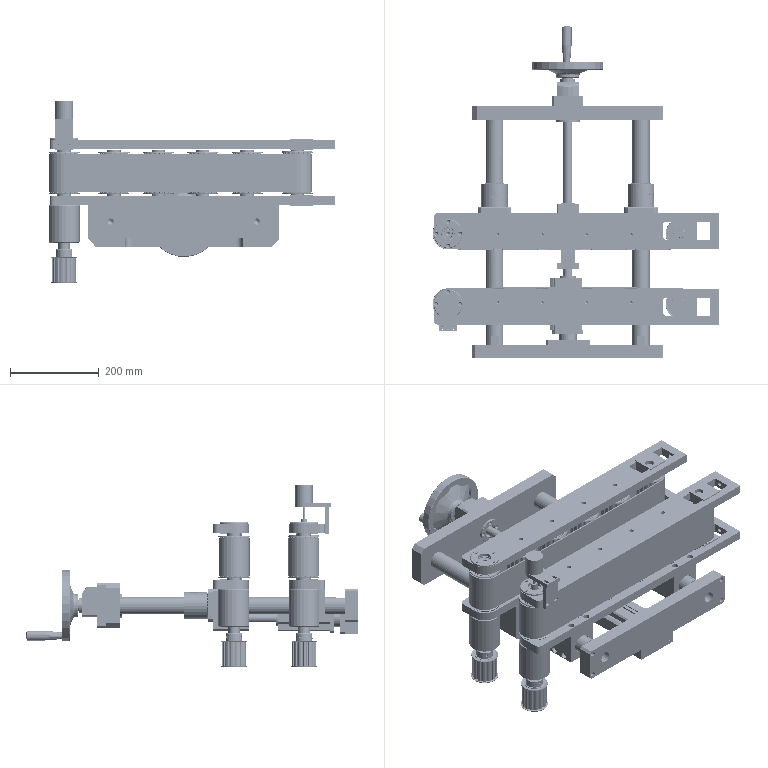Assembly | SolidWorks | mm | 131 component files | 548 solids | 15927 faces | box 646.6 x 748 x 409 mm | volume 15901574 mm3 | plane 6016 | cylinder 5265 | spline 3633 | cone 837 | torus 110 | sphere 66 | commonest cylinder face diameters 2.94 x548 2.84 x548 5.667 x216 58.13 x204 63.31 x192 0.361 x182 0.154 x168 0.628 x156
Bill of materials:
11_16X160 | 1 |  | Disc-shaped handwheel-like body: a flat circular rim with a recessed, scalloped (lobed) inner face that slopes conically down to a raised central hub. The hub has a through bore with a small keyway-like notch. A tapered cylindrical handle sticks out from the rim face, parallel to the axis.
1105_LMKPUU40 | 2 |  | Flanged cylindrical housing: a long round body with a square flange near one end. The flange has chamfered corners and four corner through-holes. The body has a large through bore. Small spherical elements are visible inside the bore, and a short stepped spigot sits on the far side of the flange.
ref7 | 1 |  | Ring-shaped rolling-element assembly: concentric inner and outer rings with a single row of spheres between them. The faces are open (no visible shields). The outer cylindrical surface is plain.
6004E-Z | 26 |  | Ring-shaped rolling-element assembly: inner and outer rings with a single row of spheres in the gap. Faces are open, and the outer edges are slightly rounded or faceted.
CounterMountingPlate | 1 |  | Thick rectangular plate with small chamfers on all four corners, one large central through-hole offset toward one end, and four small corner through-holes.
DigitalDisplay.0 | 1 |  | Block with two concave arc-shaped ends. A short cylindrical boss sticks out from one face and a smaller pin from the opposite face. The block has a through-hole and a chamfered edge.
E6B2-CWZ1XEncoder | 1 |  | Cylindrical body with a short smaller-diameter pilot step and a slender shaft coming out of one end. The shaft appears to have a flat along part of its length.
EncoderAxis | 1 |  | Stepped cylindrical pin: a larger central collar between two smaller shaft sections of different diameters. The end view shows flats or an irregular polygonal outline, and one end is lightly chamfered.
EncoderMountingSeat | 1 |  | L-shaped bracket. The horizontal plate has a rounded end with a large central hole and three small holes around it. Two slots sit near the bend, and the vertical leg has two further slots near its free end.
FixedSeat | 2 |  | Cube-like block with a large through bore. A narrow slit runs from the bore out to one edge, forming a split clamp. One face has four small holes, with countersunk/conical entries visible from the opposite face.
GuidePostMountingPlate | 1 | 1023 Carbon Steel Plate (SS) | Long rectangular bar with chamfered edges and a large through-hole near each end. The underside has a central recess/cutout between two end pads, and there is a small square window. Rows of small holes run on the top and side faces.
GuideSleeve | 2 |  | Plain thin-walled cylindrical tube with open ends, constant wall thickness, and no other features.
HandwheelEndCap | 1 |  | Thick flat annular disc (washer-like) with a single central through-hole and chamfered outer edges.
HandwheelMountingPlate | 1 |  | Elongated flat rectangular bar/plate with chamfered corners, a stepped (counterbored) central hole surrounded by four small holes in a cross pattern, and a counterbored hole near each end.
hexagon socket head cap screws gb | 4 |  | Cap-screw-shaped part: cylindrical head with hexagonal socket recess and rounded top edge, plain cylindrical shank with chamfered tip.
LimitingBlock | 1 |  | Rectangular hollow frame block with a square through-opening, chamfered outer corners, and a small hole through each side wall.
Nut | 1 |  | Long rectangular bar with a T-shaped cross-section (wider flange on one side) and a large round bore running lengthwise through it.
RisingBeltCylinderSeat | 1 |  | Two parallel rectangular plates of different size with chamfered corners, connected by a central cylindrical hub/spacer; each plate has four larger holes and four smaller corner holes.
RisingCylinderOutputPlate | 1 |  | Fork/U-shaped bracket block: base with two upright prongs forming a rectangular slot, a raised central tongue on one face, and three holes in the base (larger central hole, two side holes).
RisingCylinderSeatPlate | 1 |  | Rectangular prismatic block with two larger through-holes in one face and two small holes in an adjacent perpendicular face.
RisingGuidePost | 2 |  | Long slender cylindrical pin with a small axial hole at one end and a slight reduced-diameter step near that end.
Rolling bearings 51103 GB 301-1995 | 1 |  | Two identical flat annular rings (washers) stacked coaxially with a gap, and one circular row of equal-size spheres between them. The overall layout looks like a thrust ball bearing.
ScrewRod | 1 |  | Slender solid stepped cylindrical shaft with three diameters decreasing toward one end.
ScrewRodBearingEndCap | 1 |  | Thin flat annular ring/flange with a large central bore and four countersunk holes equally spaced on a circle.
ScrewRodFixingNut | 2 |  | Ring with a large central bore and four rectangular slots evenly spaced around the outer periphery, with chamfered edges (resembles a slotted round nut shape).
SDA50-80Cylinder | 1 |  | Prismatic body with a roughly square cross-section and chamfered corners, a through-hole at each of the four corners running the full length, and long slots on its side faces. One end face has a large circular recess, and a short cylindrical boss sticks out of the other end.
SDA50-80CylinderPiston | 1 |  | Solid round rod. One end is flat. The other end has a narrow ring-shaped groove close to the end face and a chamfer on the edge.
BearingPlate3 | 16 |  | Flat ring with a large central hole and chamfered edges on both faces.
S16-H12-01(SupportWheel) | 8 |  | Toothed cylindrical part with a flange at each end and a central through-bore. The outer surface has evenly spaced axial teeth/grooves, and the bore has an internal step.
SupportWheelAxis | 8 |  | Stepped cylindrical pin with a long main body, a short section of slightly smaller diameter, and a small-diameter spigot at one end. The larger end face has a small central hole with a conical bottom.
'-SynchronousBeltLength1260 | 2 |  | Thin-walled closed band with an obround (stadium-shaped) outline, open at both ends.
TensionAdjustmentBlock | 4 |  | Solid rectangular bar with three round through-holes in one long face: two larger holes near the ends and one smaller hole between them. The holes are not evenly spaced.
TensionBlock | 4 |  | Block with an I-shaped cross-section: wide top and bottom plates joined by a narrower central body. It has a large vertical through-hole near one corner and a small horizontal hole in one side face.
BearingPlate2 | 4 |  | Flat ring with a large central hole, square-edged with no visible chamfers.
S16-H12-01 | 2 |  | Toothed cylindrical part with a flange at each end and a central through-bore, with an internal step inside the bore. It looks the same as the part shown for unnamed part.
TractionDrivenWheelAxis | 2 |  | Solid cylindrical pin with a slightly larger diameter in the middle and short, slightly smaller-diameter sections at both ends, forming small shoulders. The end faces are flat with small chamfers.
S14H-H12-01(FrontWheel) | 2 |  | Toothed cylindrical part with a flange at each end and an extended cylindrical hub on one side. The central bore has one rectangular keyway, and the hub has at least two small radial holes.
S16-H12-01(DriveWheel) | 2 |  | Cylindrical body with axial teeth around the outside and a thin flange at each end, with a keyed through bore. It looks like a toothed pulley.
TractionDriveAxis | 2 |  | Long, thin stepped cylindrical pin or shaft. It has a larger-diameter upper section, a longer smaller-diameter lower section, and a short reduced stub at the top end with a small axial hole.
TractionDriveWheelBearingHousing | 2 |  | Thick-walled cylindrical housing with a large central bore. A shallow raised ring sits on the top face, the bore has an internal step, and four axial holes are evenly spaced around the bore.
TractionDriveWheelLimitSleeve | 2 |  | Plain thin-walled cylindrical tube or sleeve, roughly as long as its outer diameter.
TractionDriveWheelLimitSleeve2 | 2 |  | Short, thin-walled ring (spacer or collar shape) whose axial length is much smaller than its diameter.
TractionDriveWheelLimitSleeve3 | 2 |  | Short cylindrical sleeve or spacer with a thicker wall than the other plain tubes, with axial length about half its diameter.
TractionDriveWheelBearingEndCap | 2 |  | Thin circular flange plate with a large central through hole, four countersunk holes evenly spaced around it, and a shallow raised spigot or boss on one face.
TractionMachineBottomPlate | 1 |  | Rectangular bar or plate with chamfered corners. It has two larger through holes near the ends and four small holes near the corners.
WheelMountingPlateA | 1 |  | Long, flat arm plate. One end is rounded and carries a large through hole with four small holes around it. The other end has an open rectangular slot that forms two fork tines. Four holes are spaced in a line along the centerline.
WheelMountingPlateA-1 | 1 | 1023 Carbon Steel Plate (SS) | Long, flat arm plate like part-8, with a large hole and four small holes at the rounded end and a forked open slot at the other end, plus extra groups of holes along its length.
WheelMountingPlateB | 1 |  | Long, flat arm plate with a large hole and four small holes at the rounded end, four holes in a line along the centerline, and a forked open slot at the far end. It also has small holes in the side edge near the large hole.
WheelMountingPlateB-1 | 1 |  | Long, flat arm plate like part-10, with a large hole and four small holes at the rounded end and a forked open slot at the far end, plus four-hole groups near both ends.
Mates:
1. coincident | WheelMountingPlateA-1 face at (290.493, -53.411, 641) dir (0, 1, 0) | TensionBlock-1 face at (260.493, -53.411, 621) dir (0, -1, 0)
2. coincident | WheelMountingPlateA-1 face at (-24.507, -33.411, 621) dir (0, 0, -1) | TensionBlock-1 face at (260.493, -8.411, 621) dir (0, 0, 1)
3. coincident | WheelMountingPlateA-1 face at (290.493, -73.411, 621) dir (1, 0, 0) | TensionAdjustmentBlock-1 face at (290.493, -33.411, 631) dir (-1, 0, 0)
4. concentric | WheelMountingPlateA-1 face at (290.493, -3.411, 631) dir (1, 0, 0) r 3.4 | TensionAdjustmentBlock-1 face at (310.493, -3.411, 631) dir (1, 0, 0) r 7
5. concentric | WheelMountingPlateA-1 face at (290.493, -63.411, 631) dir (1, 0, 0) r 3.4 | TensionAdjustmentBlock-1 face at (310.493, -63.411, 631) dir (1, 0, 0) r 7
6. coincident | WheelMountingPlateB-1 face at (290.493, -244.411, 621) dir (1, 0, 0) | TensionAdjustmentBlock-2 face at (290.493, -204.411, 631) dir (-1, 0, 0)
7. coincident | WheelMountingPlateB-1 face at (290.493, -224.411, 641) dir (0, 1, 0) | TensionBlock-3 face at (260.493, -224.411, 641) dir (0, -1, 0)
8. concentric | WheelMountingPlateB-1 face at (290.493, -174.411, 631) dir (1, 0, 0) r 3.4 | TensionAdjustmentBlock-2 face at (310.493, -174.411, 631) dir (1, 0, 0) r 7
9. concentric | WheelMountingPlateB-1 face at (290.493, -234.411, 631) dir (1, 0, 0) r 3.4 | TensionAdjustmentBlock-2 face at (310.493, -234.411, 631) dir (1, 0, 0) r 7
10. concentric | TractionMachineBottomPlate-1 face at (-194.507, -319.411, 458) dir (0, 1, 0) r 20 | RisingGuidePost-1 face at (-194.507, 225.589, 458) dir (0, -1, 0) r 20
11. distance | TractionMachineBottomPlate-1 face at (-244.507, -319.411, 495.5) dir (0, -1, 0) | RisingGuidePost-1 face at (-194.507, -294.411, 458) dir (0, -1, 0)
12. concentric | TractionMachineBottomPlate-1 face at (135.493, -319.411, 458) dir (0, 1, 0) r 20 | RisingGuidePost-2 face at (135.493, 225.589, 458) dir (0, -1, 0) r 20
13. distance | TractionMachineBottomPlate-1 face at (-244.507, -319.411, 495.5) dir (0, -1, 0) | RisingGuidePost-2 face at (135.493, -294.411, 458) dir (0, -1, 0)
14. concentric | RisingGuidePost-1 face at (-194.507, 225.589, 458) dir (0, -1, 0) r 20 | FixedSeat-1 face at (-194.507, -244.411, 458) dir (0, 1, 0) r 20
15. parallel | TractionMachineBottomPlate-1 face at (-29.507, -304.411, 420.5) dir (0, 0, -1) | FixedSeat-1 face at (-194.507, -206.911, 423) dir (0, 0, -1)
16. concentric | RisingGuidePost-2 face at (135.493, 225.589, 458) dir (0, -1, 0) r 20 | FixedSeat-2 face at (135.493, -169.411, 458) dir (0, -1, 0) r 20
17. coincident | FixedSeat-1 face at (-194.507, -206.911, 423) dir (0, 0, -1) | FixedSeat-2 face at (135.493, -206.911, 423) dir (0, 0, -1)
18. coincident | TractionMachineBottomPlate-1 face at (-244.507, -289.411, 495.5) dir (0, 1, 0) | RisingBeltCylinderSeat-1 face at (-29.507, -289.411, 430.5) dir (0, -1, 0)
19. width | RisingBeltCylinderSeat-1 face at (20.493, -279.411, 393) dir (1, 0, 0) | RisingBeltCylinderSeat-1 face at (-79.507, -279.411, 393) dir (-1, 0, 0) | TractionMachineBottomPlate-1 face at (-244.507, -289.411, 495.5) dir (-1, 0, 0) | TractionMachineBottomPlate-1 face at (185.493, -289.411, 495.5) dir (1, 0, 0)
20. concentric | RisingGuidePost-2 face at (135.493, 225.589, 458) dir (0, -1, 0) r 20 | GuidePostMountingPlate-1 face at (135.493, -66.411, 458) dir (0, 1, 0) r 22
21. concentric | RisingGuidePost-1 face at (-194.507, 225.589, 458) dir (0, -1, 0) r 20 | GuidePostMountingPlate-1 face at (-194.507, -66.411, 458) dir (0, 1, 0) r 22
22. coincident | GuidePostMountingPlate-1 face at (-14.507, -69.411, 443) dir (0, 0, 1) | Nut-1 face at (-54.507, -104.411, 443) dir (0, 0, -1)
23. coincident | GuidePostMountingPlate-1 face at (-44.507, -69.411, 473) dir (1, 0, 0) | Nut-1 face at (-44.507, 30.589, 473) dir (-1, 0, 0)
24. width | RisingCylinderOutputPlate-1 face at (-57.007, -43.411, 468) dir (1, 0, 0) | RisingCylinderOutputPlate-1 face at (-2.007, -43.411, 468) dir (-1, 0, 0) | Nut-1 face at (-54.507, -104.411, 443) dir (-1, 0, 0) | Nut-1 face at (-4.507, -104.411, 443) dir (1, 0, 0)
25. coincident | GuidePostMountingPlate-1 face at (102.993, -28.411, 475) dir (0, -1, 0) | RisingCylinderOutputPlate-1 face at (-29.507, -28.411, 428) dir (0, 1, 0)
26. concentric | RisingGuidePost-1 face at (-194.507, 225.589, 458) dir (0, -1, 0) r 20 | HandwheelMountingPlate-1 face at (-194.507, 217.589, 458) dir (0, 1, 0) r 20
27. concentric | RisingGuidePost-2 face at (135.493, 225.589, 458) dir (0, -1, 0) r 20 | HandwheelMountingPlate-1 face at (135.493, 247.589, 458) dir (0, 1, 0) r 12
28. coincident | RisingGuidePost-2 face at (135.493, 225.589, 458) dir (0, 1, 0) | HandwheelMountingPlate-1 face at (135.493, 225.589, 458) dir (0, -1, 0)
29. coincident | WheelMountingPlateB-1 face at (-24.507, -204.411, 621) dir (0, 0, -1) | TensionBlock-3 face at (260.493, -179.411, 621) dir (0, 0, 1)
30. concentric | TensionBlock-3 face at (225.493, -197.911, 618.5) dir (0, 0, 1) r 9.5 | TractionDrivenWheel-1/6004E-Z-1 face at (225.493, -197.911, 527) dir (0, 0, 1) r 10
31. coincident | WheelMountingPlateB-1 plane at (225.493, -204.411, 631) dir (1, 0, 0) | TractionDrivenWheel-1/TractionDrivenWheelAxis-1 plane at (225.493, -197.911, 568.5) dir (-1, 0, 0)
32. coincident | 6004E-Z-1 face at (-299.852, -27.028, 624) dir (0, 0, -1) | TractionDriveWheelAssembly-1/TractionDriveAxis-1 face at (-299.507, -29.911, 624) dir (0, 0, 1)
33. concentric | 6004E-Z-1 face at (-299.507, -39.911, 630) dir (0, 0, -1) r 10 | TractionDriveWheelAssembly-1/TractionDriveAxis-1 face at (-299.507, -39.911, 965.247) dir (0, 0, 1) r 10
34. concentric | WheelMountingPlateB-1 face at (-299.507, -197.911, 641) dir (0, 0, -1) r 21 | 6004E-Z-2 face at (-299.507, -197.911, 631) dir (0, 0, 1) r 21
35. concentric | HandwheelMountingPlate-1 face at (-29.507, 217.589, 458) dir (0, 1, 0) r 10 | 11_16X160-1 face at (-29.507, 309.589, 458) dir (0, -1, 0) r 8
36. concentric | HandwheelMountingPlate-1 face at (-29.507, 217.589, 458) dir (0, 1, 0) r 10 | DigitalDisplay.0-1 face at (-29.507, 309.589, 458) dir (0, -1, 0) r 17
37. width | CounterMountingPlate-1 face at (-64.507, 269.589, 508) dir (0, 0, 1) | CounterMountingPlate-1 face at (-64.507, 269.589, 408) dir (0, 0, -1) | HandwheelMountingPlate-1 face at (185.493, 247.589, 408) dir (0, 0, -1) | HandwheelMountingPlate-1 face at (185.493, 247.589, 508) dir (0, 0, 1)
38. width | DigitalDisplay.0-1 face at (-53.507, 301.589, 437) dir (-1, 0, 0) | DigitalDisplay.0-1 face at (-5.507, 301.589, 437) dir (1, 0, 0) | CounterMountingPlate-1 face at (5.493, 269.589, 408) dir (1, 0, 0) | CounterMountingPlate-1 face at (-64.507, 269.589, 408) dir (-1, 0, 0)
39. coincident | 11_16X160-1 face at (-29.507, 309.589, 458) dir (0, -1, 0) | DigitalDisplay.0-1 face at (-29.507, 309.589, 458) dir (0, 1, 0)
40. concentric | ScrewRod-1 face at (-29.507, 267.589, 458) dir (0, -1, 0) r 8.35 | ScrewRodFixingNut-1 face at (-29.507, 255.589, 458) dir (0, -1, 0) r 8.5
41. coincident | HandwheelMountingPlate-1 face at (-29.507, 247.589, 458) dir (0, 1, 0) | CounterMountingPlate-1 face at (-29.507, 247.589, 458) dir (0, -1, 0)
42. coincident | DigitalDisplay.0-1 face at (-29.507, 269.589, 492.1) dir (0, -1, 0) | CounterMountingPlate-1 face at (-29.507, 269.589, 458) dir (0, 1, 0)
43. coincident | 11_16X160-1 face at (-32.409, 309.589, 447.806) dir (0.9992, 0, -0.03922) | ScrewRod-1 face at (-32.593, 304.589, 443.11) dir (0.9992, 0, -0.03922)
44. coincident | 11_16X160-1 face at (-30.585, 329.589, 430.521) dir (0, 1, 0) | HandwheelEndCap-1 face at (-29.507, 329.589, 458) dir (0, -1, 0)
45. concentric | ScrewRod-1 face at (-29.507, 327.589, 458) dir (0, 1, 0) r 2.5 | HandwheelEndCap-1 face at (-29.507, 329.589, 458) dir (0, 1, 0) r 3.5
46. concentric | ScrewRod-1 face at (-29.507, -441.983, 458) dir (0, -1, 0) r 10 | ScrewRodBearingEndCap-1 face at (-29.507, 217.589, 458) dir (0, -1, 0) r 14.5
47. coincident | HandwheelMountingPlate-1 face at (-29.507, 217.589, 458) dir (0, -1, 0) | ScrewRodBearingEndCap-1 face at (-29.507, 217.589, 458) dir (0, 1, 0)
48. concentric | HandwheelMountingPlate-1 face at (-29.507, 217.589, 479) dir (0, -1, 0) r 1.65 | ScrewRodBearingEndCap-1 face at (-29.507, 212.589, 479) dir (0, -1, 0) r 2.25
49. coincident | HandwheelMountingPlate-1 face at (-29.507, 238.589, 458) dir (0, 1, 0) | Rolling bearings 51103 GB 301-1995-1 face at (-37.584, 238.589, 454.031) dir (0, -1, 0)
50. concentric | HandwheelMountingPlate-1 face at (-29.507, 238.589, 458) dir (0, 1, 0) r 15 | Rolling bearings 51103 GB 301-1995-1 face at (-29.507, 234.363, 458) dir (0, -1, 0) r 8.5
51. coincident | Rolling bearings 51103 GB 301-1995-1 face at (-37.136, 247.589, 454.252) dir (0, 1, 0) | ScrewRodFixingNut-1 face at (-29.507, 247.589, 458) dir (0, -1, 0)
52. distance | ScrewRod-1 face at (-29.507, -82.411, 458) dir (0, -1, 0) | Nut-1 face at (-29.507, -119.411, 458) dir (0, -1, 0)
53. coincident | TractionMachineBottomPlate-1 face at (-29.507, -304.411, 420.5) dir (0, 0, -1) | RisingCylinderSeatPlate-1 face at (20.493, -289.411, 420.5) dir (0, 0, 1)
54. coincident | TractionMachineBottomPlate-1 face at (-244.507, -319.411, 495.5) dir (0, -1, 0) | RisingCylinderSeatPlate-1 face at (-29.507, -319.411, 406.75) dir (0, -1, 0)
55. width | RisingCylinderSeatPlate-1 face at (20.493, -289.411, 420.5) dir (1, 0, 0) | RisingCylinderSeatPlate-1 face at (-79.507, -289.411, 420.5) dir (-1, 0, 0) | TractionMachineBottomPlate-1 face at (-244.507, -289.411, 495.5) dir (-1, 0, 0) | TractionMachineBottomPlate-1 face at (185.493, -289.411, 495.5) dir (1, 0, 0)
56. concentric | RisingGuidePost-2 face at (135.493, 225.589, 458) dir (0, -1, 0) r 20 | 1105_LMKPUU40-1 face at (135.493, 47.467, 458) dir (0, 1, 0) r 30
57. coincident | GuidePostMountingPlate-1 face at (-232.007, 6.589, 400) dir (0, 1, 0) | 1105_LMKPUU40-1 face at (114.492, 6.589, 479.001) dir (0, -1, 0)
58. parallel | GuidePostMountingPlate-1 face at (172.993, -73.411, 400) dir (1, 0, 0) | 1105_LMKPUU40-1 face at (172.993, 6.589, 458) dir (1, 0, 0)
59. coincident | GuidePostMountingPlate-1 face at (135.493, -6.411, 458) dir (0, 1, 0) | GuideSleeve-1 face at (135.493, -6.411, 458) dir (0, 1, 0)
60. concentric | GuidePostMountingPlate-1 face at (135.493, -66.411, 458) dir (0, 1, 0) r 22 | GuideSleeve-1 face at (135.493, -6.411, 458) dir (0, -1, 0) r 22
61. coincident | Nut-1 face at (-54.507, -104.411, 473) dir (0, 0, 1) | LimitingBlock-1 face at (-44.507, 26.589, 473) dir (0, 0, -1)
62. coincident | Nut-1 face at (-14.507, 30.589, 473) dir (1, 0, 0) | LimitingBlock-1 face at (-14.507, 26.589, 443) dir (-1, 0, 0)
63. distance | Nut-1 face at (-29.507, 30.589, 458) dir (0, 1, 0) | LimitingBlock-1 face at (-29.507, 26.589, 458) dir (0, 1, 0)
64. coincident | FixedSeat-1 face at (-159.507, -244.411, 423) dir (0, -1, 0) | FixedSeat-2 face at (100.493, -244.411, 423) dir (0, -1, 0)
65. distance | GuidePostMountingPlate-1 face at (-232.007, -73.411, 400) dir (0, -1, 0) | FixedSeat-1 face at (-159.507, -169.411, 423) dir (0, 1, 0)
66. concentric | SDA50-80Cylinder-1 face at (-29.507, -205.411, 430.5) dir (0, 1, 0) r 10 | SDA50-80CylinderPiston-1 face at (-29.507, -149.411, 430.5) dir (0, 1, 0) r 10
67. distance | RisingCylinderOutputPlate-1 face at (-29.507, -43.411, 441.5) dir (0, 0, 1) | Nut-1 face at (-54.507, -104.411, 443) dir (0, 0, -1)
68. concentric | RisingCylinderOutputPlate-1 face at (-29.507, -28.411, 430.5) dir (0, 1, 0) r 5.5 | SDA50-80CylinderPiston-1 face at (-29.507, -149.411, 430.5) dir (0, 1, 0) r 10
69. coincident | RisingCylinderOutputPlate-1 face at (-29.507, -49.411, 430.5) dir (0, -1, 0) | SDA50-80CylinderPiston-1 face at (-29.507, -49.411, 430.5) dir (0, 1, 0)
70. concentric | RisingBeltCylinderSeat-1 face at (-53.507, -266.411, 406.5) dir (0, -1, 0) r 4.5 | SDA50-80Cylinder-1 face at (-53.507, -249.411, 406.5) dir (0, -1, 0) r 5.5
71. concentric | TensionAdjustmentBlock-1 face at (290.493, -39.911, 631) dir (1, 0, 0) r 4.1 | hexagon socket head cap screws gb-6 face at (304.493, -39.911, 631) dir (1, 0, 0) r 0.8
72. concentric | TensionAdjustmentBlock-2 face at (290.493, -197.911, 631) dir (1, 0, 0) r 4.1 | hexagon socket head cap screws gb-7 face at (304.493, -197.911, 631) dir (1, 0, 0) r 0.8
73. concentric | ScrewRodBearingEndCap-1 face at (-29.507, 217.589, 458) dir (0, -1, 0) r 27 | -6003-1 face at (-29.507, 231.299, 458) dir (0, 1, 0) r 17.5
74. coincident | ScrewRod-1 face at (-39.499, 217.589, 458.392) dir (0, 1, 0) | -6003-1 face at (-12.007, 217.589, 458) dir (0, -1, 0)
75. coincident | HandwheelMountingPlate-1 face at (-29.507, 227.589, 458) dir (0, -1, 0) | -6003-1 face at (-12.007, 227.589, 458) dir (0, 1, 0)
76. coincident | ScrewRodFixingNut-1 face at (-29.507, 255.589, 458) dir (0, 1, 0) | ScrewRodFixingNut-6 face at (-29.507, 255.589, 458) dir (0, -1, 0)
77. concentric | ScrewRod-1 face at (-29.507, 267.589, 458) dir (0, -1, 0) r 8.35 | ScrewRodFixingNut-6 face at (-29.507, 263.589, 458) dir (0, -1, 0) r 8.5
78. distance | EncoderAxis-1 face at (-293.716, -193.145, 654) dir (0, 0, 1) | TractionDriveWheelAssembly-2/TractionDriveAxis-1 face at (-299.507, -197.911, 636) dir (0, 0, 1)
79. concentric | TractionDriveWheelAssembly-2/TractionDriveAxis-1 face at (-299.507, -197.911, 636) dir (0, 0, 1) r 5 | EncoderAxis-1 face at (-299.507, -197.911, 814.656) dir (0, 0, 1) r 5
80. concentric | E6B2-CWZ1XEncoder-1 face at (-299.507, -182.911, 690) dir (0, 0, -1) r 1.25 | EncoderMountingSeat-1 face at (-299.507, -182.911, 683) dir (0, 0, -1) r 3.5
81. concentric | E6B2-CWZ1XEncoder-1 face at (-286.516, -205.411, 690) dir (0, 0, -1) r 1.25 | EncoderMountingSeat-1 face at (-286.516, -205.411, 683) dir (0, 0, -1) r 3.5
82. coincident | E6B2-CWZ1XEncoder-1 face at (-299.507, -197.911, 690) dir (0, 0, -1) | EncoderMountingSeat-1 face at (-299.507, -197.911, 690) dir (0, 0, 1)
83. distance | TensionBlock-1 face at (210.493, -58.411, 618.5) dir (-1, 0, 0) | WheelMountingPlateA-1 face at (185.493, -13.411, 641) dir (1, 0, 0)
84. coincident | TensionAdjustmentBlock-1 face at (310.493, -33.411, 631) dir (1, 0, 0) | hexagon socket head cap screws gb-6 face at (310.493, -39.911, 631) dir (-1, 0, 0)
85. coincident | WheelMountingPlateA-1-1 plane at (-24.507, -33.411, 505) dir (0, 1, 0) | GuidePostMountingPlate-1 plane at (-29.507, -33.411, 447.5) dir (0, 1, 0)
86. coincident | WheelMountingPlateA-1-1 face at (-24.507, -33.411, 495) dir (0, 0, -1) | GuidePostMountingPlate-1 face at (-29.507, -33.411, 495) dir (0, 0, 1)
87. concentric | WheelMountingPlateA-1-1 face at (82.993, -8.411, 515) dir (0, 0, 1) r 5.5 | GuidePostMountingPlate-1 face at (82.993, -8.411, 495) dir (0, 0, 1) r 4.25
88. concentric | WheelMountingPlateA-1-1 face at (-299.507, -39.911, 515) dir (0, 0, -1) r 23 | TractionDriveWheelAssembly-1/TractionDriveWheelLimitSleeve-1 face at (-299.507, -39.911, 520) dir (0, 0, -1) r 15
89. coincident | WheelMountingPlateA-1-1 face at (-24.507, -33.411, 495) dir (0, 0, -1) | TractionDriveWheelAssembly-1/TractionDriveWheelBearingHousing-2 face at (-320.507, -39.911, 495) dir (0, 0, 1)
90. coincident | WheelMountingPlateA-1 plane at (-24.507, -33.411, 631) dir (-1, 0, 0) | WheelMountingPlateA-1-1 plane at (-24.507, -33.411, 505) dir (-1, 0, 0)
91. coincident | WheelMountingPlateA-1 plane at (-24.507, -33.411, 631) dir (0, 1, 0) | WheelMountingPlateA-1-1 plane at (-24.507, -33.411, 505) dir (0, 1, 0)
92. distance | WheelMountingPlateA-1 face at (-24.507, -33.411, 641) dir (0, 0, 1) | WheelMountingPlateA-1-1 face at (-24.507, -33.411, 495) dir (0, 0, -1)
93. concentric | WheelMountingPlateA-1 face at (-299.507, -12.911, 621) dir (0, 0, -1) r 1.65 | TractionDriveWheelBearingEndCap-1 face at (-299.507, -12.911, 646) dir (0, 0, 1) r 2.25
94. concentric | WheelMountingPlateA-1 face at (-299.507, -66.911, 621) dir (0, 0, -1) r 1.65 | TractionDriveWheelBearingEndCap-1 face at (-299.507, -66.911, 646) dir (0, 0, 1) r 2.25
95. coincident | WheelMountingPlateA-1 face at (-24.507, -33.411, 641) dir (0, 0, 1) | TractionDriveWheelBearingEndCap-1 face at (-299.507, -7.411, 641) dir (0, 0, -1)
96. coincident | WheelMountingPlateA-1-1 face at (290.493, -13.411, 515) dir (0, -1, 0) | TensionBlock-7 face at (260.493, -13.411, 495) dir (0, 1, 0)
97. width | TensionBlock-7 face at (235.493, -33.411, 492.5) dir (0, 0, -1) | TensionBlock-7 face at (235.493, -33.411, 517.5) dir (0, 0, 1) | WheelMountingPlateA-1-1 face at (-24.507, -33.411, 515) dir (0, 0, 1) | WheelMountingPlateA-1-1 face at (-24.507, -33.411, 495) dir (0, 0, -1)
98. coincident | TensionBlock-1 face at (260.493, -58.411, 618.5) dir (1, 0, 0) | TensionBlock-7 face at (260.493, -58.411, 492.5) dir (1, 0, 0)
99. concentric | WheelMountingPlateA-1-1 face at (290.493, -3.411, 505) dir (1, 0, 0) r 3.4 | TensionAdjustmentBlock-5 face at (310.493, -3.411, 505) dir (1, 0, 0) r 7
100. concentric | WheelMountingPlateA-1-1 face at (290.493, -63.411, 505) dir (1, 0, 0) r 3.4 | TensionAdjustmentBlock-5 face at (310.493, -63.411, 505) dir (1, 0, 0) r 4.5
101. coincident | WheelMountingPlateA-1-1 face at (290.493, -73.411, 495) dir (1, 0, 0) | TensionAdjustmentBlock-5 face at (290.493, -33.411, 505) dir (-1, 0, 0)
102. concentric | TensionAdjustmentBlock-5 face at (290.493, -39.911, 505) dir (1, 0, 0) r 4.1 | hexagon socket head cap screws gb-8 face at (304.493, -39.911, 505) dir (1, 0, 0) r 0.8
103. coincident | TensionAdjustmentBlock-5 face at (310.493, -33.411, 505) dir (1, 0, 0) | hexagon socket head cap screws gb-8 face at (310.493, -39.911, 505) dir (-1, 0, 0)
104. concentric | TractionDrivenWheel-2/TractionDrivenWheelAxis-1 face at (225.493, -39.911, 520) dir (0, 0, -1) r 9.5 | TensionBlock-7 face at (225.493, -39.911, 517.5) dir (0, 0, -1) r 9.5
105. coincident | TractionDrivenWheel-2/BearingPlate2-2 face at (225.493, -39.911, 517.5) dir (0, 0, -1) | TensionBlock-7 face at (235.493, -33.411, 517.5) dir (0, 0, 1)
106. concentric | WheelMountingPlateA-1-1 face at (-187.007, -42.411, 495) dir (0, 0, -1) r 6 | SupportWheelAssembly-2/SupportWheelAxis-1 face at (-187.007, -42.411, 496) dir (0, 0, 1) r 6
107. concentric | WheelMountingPlateA-1-1 face at (112.993, -42.411, 495) dir (0, 0, -1) r 6 | SupportWheelAssembly-2/SupportWheelAxis-4 face at (112.993, -42.411, 496) dir (0, 0, 1) r 6
108. coincident | WheelMountingPlateA-1-1 face at (-24.507, -33.411, 515) dir (0, 0, 1) | SupportWheelAssembly-2/BearingPlate3-4 face at (112.993, -42.411, 515) dir (0, 0, -1)
109. coincident | TensionAdjustmentBlock-2 face at (310.493, -204.411, 631) dir (1, 0, 0) | hexagon socket head cap screws gb-7 face at (310.493, -197.911, 631) dir (-1, 0, 0)
110. distance | FixedSeat-1 face at (-159.507, -244.411, 423) dir (0, -1, 0) | TractionMachineBottomPlate-1 face at (-244.507, -289.411, 495.5) dir (0, 1, 0)
111. concentric | WheelMountingPlateB-1-1 face at (-218.507, -178.911, 515) dir (0, 0, 1) r 4.5 | FixedSeat-1 face at (-218.507, -178.911, 495) dir (0, 0, 1) r 3.4
112. concentric | WheelMountingPlateB-1-1 face at (-170.507, -178.911, 515) dir (0, 0, 1) r 4.5 | FixedSeat-1 face at (-170.507, -178.911, 495) dir (0, 0, 1) r 3.4
113. coincident | WheelMountingPlateB-1-1 face at (-24.507, -204.411, 495) dir (0, 0, -1) | FixedSeat-1 face at (-194.507, -206.911, 495) dir (0, 0, 1)
114. concentric | WheelMountingPlateB-1-1 face at (-299.507, -197.911, 515) dir (0, 0, -1) r 22.5 | TractionDriveWheelAssembly-2/TractionDriveWheelLimitSleeve-1 face at (-299.507, -197.911, 520) dir (0, 0, -1) r 15
115. coincident | WheelMountingPlateB-1-1 face at (-24.507, -204.411, 495) dir (0, 0, -1) | TractionDriveWheelAssembly-2/TractionDriveWheelBearingHousing-2 face at (-299.507, -176.911, 495) dir (0, 0, 1)
116. concentric | WheelMountingPlateB-1-1 face at (-299.507, -169.911, 515) dir (0, 0, 1) r 2.5 | TractionDriveWheelAssembly-2/TractionDriveWheelBearingHousing-2 face at (-299.507, -169.911, 410) dir (0, 0, -1) r 3.5
117. concentric | WheelMountingPlateA-1-1 face at (-299.507, -11.911, 515) dir (0, 0, 1) r 2.5 | TractionDriveWheelAssembly-1/TractionDriveWheelBearingHousing-2 face at (-299.507, -11.911, 410) dir (0, 0, -1) r 3.5
118. coincident | WheelMountingPlateB-1 plane at (-24.507, -204.411, 631) dir (-1, 0, 0) | WheelMountingPlateB-1-1 plane at (-24.507, -204.411, 505) dir (-1, 0, 0)
119. coincident | WheelMountingPlateB-1 plane at (-24.507, -204.411, 631) dir (0, 1, 0) | WheelMountingPlateB-1-1 plane at (-24.507, -204.411, 505) dir (0, 1, 0)
120. distance | WheelMountingPlateB-1 face at (-24.507, -204.411, 641) dir (0, 0, 1) | WheelMountingPlateB-1-1 face at (-24.507, -204.411, 495) dir (0, 0, -1)
121. concentric | WheelMountingPlateB-1 face at (-299.507, -170.911, 621) dir (0, 0, -1) r 1.65 | TractionDriveWheelBearingEndCap-2 face at (-299.507, -170.911, 646) dir (0, 0, 1) r 2.25
122. concentric | WheelMountingPlateB-1 face at (-299.507, -224.911, 621) dir (0, 0, -1) r 1.65 | TractionDriveWheelBearingEndCap-2 face at (-299.507, -224.911, 646) dir (0, 0, 1) r 2.25
123. coincident | WheelMountingPlateB-1 face at (-24.507, -204.411, 641) dir (0, 0, 1) | TractionDriveWheelBearingEndCap-2 face at (-267.007, -197.911, 641) dir (0, 0, -1)
124. concentric | E6B2-CWZ1XEncoder-1 face at (-299.507, -197.911, 690) dir (0, 0, 1) r 20 | EncoderAxis-1 face at (-299.507, -197.911, 814.656) dir (0, 0, 1) r 3
125. coincident | E6B2-CWZ1XEncoder-1 face at (-299.507, -197.911, 670) dir (0, 0, -1) | EncoderAxis-1 face at (-297.19, -196.005, 670) dir (0, 0, 1)
126. coincident | WheelMountingPlateB-1 face at (-339.507, -244.411, 621) dir (0, -1, 0) | EncoderMountingSeat-1 face at (-279.507, -244.411, 620) dir (0, 1, 0)
127. coincident | TensionBlock-3 face at (235.493, -204.411, 618.5) dir (0, 0, -1) | TractionDrivenWheel-1/BearingPlate2-2 face at (225.493, -197.911, 618.5) dir (0, 0, 1)
128. concentric | WheelMountingPlateB-1-1 face at (-187.007, -195.411, 495) dir (0, 0, -1) r 6 | SupportWheelAssembly-1/SupportWheelAxis-1 face at (-187.007, -195.411, 496) dir (0, 0, 1) r 6
129. concentric | WheelMountingPlateB-1-1 face at (112.993, -195.411, 495) dir (0, 0, -1) r 6 | SupportWheelAssembly-1/SupportWheelAxis-4 face at (112.993, -195.411, 496) dir (0, 0, 1) r 6
130. coincident | WheelMountingPlateB-1-1 face at (-24.507, -204.411, 515) dir (0, 0, 1) | SupportWheelAssembly-1/BearingPlate3-4 face at (112.993, -195.411, 515) dir (0, 0, -1)
131. coincident | WheelMountingPlateB-1-1 face at (290.493, -184.411, 515) dir (0, -1, 0) | TensionBlock-8 face at (260.493, -184.411, 515) dir (0, 1, 0)
132. width | TensionBlock-8 face at (235.493, -204.411, 492.5) dir (0, 0, -1) | TensionBlock-8 face at (235.493, -204.411, 517.5) dir (0, 0, 1) | WheelMountingPlateB-1-1 face at (-24.507, -204.411, 515) dir (0, 0, 1) | WheelMountingPlateB-1-1 face at (-24.507, -204.411, 495) dir (0, 0, -1)
133. coincident | TensionBlock-3 face at (260.493, -179.411, 643.5) dir (1, 0, 0) | TensionBlock-8 face at (260.493, -179.411, 517.5) dir (1, 0, 0)
134. concentric | WheelMountingPlateB-1-1 face at (290.493, -174.411, 505) dir (1, 0, 0) r 3.4 | TensionAdjustmentBlock-6 face at (310.493, -174.411, 505) dir (1, 0, 0) r 7
135. concentric | WheelMountingPlateB-1-1 face at (290.493, -234.411, 505) dir (1, 0, 0) r 3.4 | TensionAdjustmentBlock-6 face at (310.493, -234.411, 505) dir (1, 0, 0) r 7
136. coincident | WheelMountingPlateB-1-1 face at (290.493, -244.411, 495) dir (1, 0, 0) | TensionAdjustmentBlock-6 face at (290.493, -204.411, 505) dir (-1, 0, 0)
137. concentric | TensionAdjustmentBlock-6 face at (290.493, -197.911, 505) dir (1, 0, 0) r 4.1 | hexagon socket head cap screws gb-9 face at (304.493, -197.911, 505) dir (1, 0, 0) r 0.8
138. coincident | TensionAdjustmentBlock-6 face at (310.493, -204.411, 505) dir (1, 0, 0) | hexagon socket head cap screws gb-9 face at (310.493, -197.911, 505) dir (-1, 0, 0)
139. coincident | RisingBeltCylinderSeat-1 face at (-29.507, -256.411, 430.5) dir (0, 1, 0) | SDA50-80Cylinder-1 face at (6.465, -256.411, 600.874) dir (0, -1, 0)
140. coincident | TractionDriveWheelBearingEndCap-2 face at (-278.507, -197.911, 637) dir (0, 0, -1) | 6004E-Z-2 face at (-280.981, -201.393, 637) dir (0, 0, 1)
141. concentric | SupportWheelAxis-1 face at (-6.386, 0.2376, 181) dir (0, 0, -1) r 10 | BearingPlate3-1 face at (-6.386, 0.2376, 81) dir (0, 0, -1) r 10.1
142. coincident | SupportWheelAxis-1 face at (-6.386, 0.2376, 76) dir (0, 0, -1) | BearingPlate3-1 face at (-6.386, 0.2376, 76) dir (0, 0, -1)
143. concentric | SupportWheelAxis-1 face at (-6.386, 0.2376, 181) dir (0, 0, -1) r 10 | S16-H12-01(SupportWheel)-1 face at (-6.386, 0.2376, 81) dir (0, 0, 1) r 17.5
144. concentric | S16-H12-01(SupportWheel)-1 face at (-6.386, 0.2376, 93) dir (0, 0, -1) r 21 | 6004E-Z-1 face at (-6.386, 0.2376, 87) dir (0, 0, 1) r 21
145. coincident | S16-H12-01(SupportWheel)-1 face at (-6.386, 0.2376, 93) dir (0, 0, -1) | 6004E-Z-1 face at (-6.386, 13.125, 93) dir (0, 0, 1)
146. coincident | BearingPlate3-1 face at (-6.386, 0.2376, 81) dir (0, 0, 1) | 6004E-Z-1 face at (-6.386, 14.088, 81) dir (0, 0, -1)
147. concentric | SupportWheelAxis-1 face at (-6.386, 0.2376, 181) dir (0, 0, -1) r 10 | 6004E-Z-5 face at (-6.386, 0.2376, 170) dir (0, 0, -1) r 21
148. coincident | S16-H12-01(SupportWheel)-1 face at (-6.386, 0.2376, 164) dir (0, 0, 1) | 6004E-Z-5 face at (-1.45, -11.667, 164) dir (0, 0, -1)
149. concentric | SupportWheelAxis-1 face at (-6.386, 0.2376, 181) dir (0, 0, -1) r 10 | BearingPlate3-5 face at (-6.386, 0.2376, 181) dir (0, 0, -1) r 15.1
150. coincident | 6004E-Z-5 face at (-1.081, -12.556, 176) dir (0, 0, 1) | BearingPlate3-5 face at (-6.386, 0.2376, 176) dir (0, 0, -1)
151. coincident | -SynchronousBeltLength1260-1 plane at (143.614, -2.262, 128.5) dir (1, 0, 0) | SupportWheelAssembly plane at (143.614, 0, 0) dir (1, 0, 0)
152. coincident | SupportWheelAxis-1 plane at (-6.386, 0.2376, 128.5) dir (0, 1, 0) | -SynchronousBeltLength1260-1 plane at (-118.886, 0.2376, 128.5) dir (0, -1, 0)
153. coincident | SupportWheelAxis-1 plane at (-6.386, 0.2376, 128.5) dir (0, 0, 1) | -SynchronousBeltLength1260-1 plane at (-118.886, -2.262, 128.5) dir (0, 0, -1)
154. concentric | S16-H12-01-1 face at (-27.031, -1.559, 128) dir (0, 0, 1) r 21 | 6004E-Z-1 face at (-27.031, -1.559, 134) dir (0, 0, -1) r 21
155. coincident | S16-H12-01-1 face at (-27.031, -1.559, 128) dir (0, 0, 1) | 6004E-Z-1 face at (-27.376, 11.323, 128) dir (0, 0, -1)
156. coincident | S16-H12-01-1 face at (-27.031, -1.559, 57) dir (0, 0, -1) | 6004E-Z-2 face at (-31.646, 10.473, 57) dir (0, 0, 1)
157. concentric | S16-H12-01-1 face at (-27.031, -1.559, 57) dir (0, 0, -1) r 21 | 6004E-Z-2 face at (-27.031, -1.559, 51) dir (0, 0, 1) r 21
158. concentric | 6004E-Z-1 face at (-27.031, -1.559, 134) dir (0, 0, -1) r 10 | TractionDrivenWheelAxis-1 face at (-27.031, -1.559, 25) dir (0, 0, 1) r 10
159. coincident | 6004E-Z-1 face at (-27.402, 12.286, 140) dir (0, 0, 1) | TractionDrivenWheelAxis-1 face at (-27.031, -1.559, 140) dir (0, 0, 1)
160. coincident | 6004E-Z-1 face at (-27.402, 12.286, 140) dir (0, 0, 1) | BearingPlate2-1 face at (-27.031, -1.559, 140) dir (0, 0, -1)
161. concentric | TractionDrivenWheelAxis-1 face at (-27.031, -1.559, 140) dir (0, 0, 1) r 9.5 | BearingPlate2-1 face at (-27.031, -1.559, 142.5) dir (0, 0, -1) r 14.6
162. concentric | TractionDrivenWheelAxis-1 face at (-27.031, -1.559, 45) dir (0, 0, -1) r 9.5 | BearingPlate2-2 face at (-27.031, -1.559, 45) dir (0, 0, -1) r 9.6
163. coincident | 6004E-Z-2 face at (-31.991, 11.372, 45) dir (0, 0, -1) | BearingPlate2-2 face at (-27.031, -1.559, 45) dir (0, 0, 1)
164. concentric | S16-H12-01(DriveWheel)-1 face at (31.813, -6.862, 45) dir (0, 0, 1) r 12.5 | TractionDriveAxis-1 face at (31.813, -6.862, 490.247) dir (0, 0, 1) r 12.5
165. distance | S16-H12-01(DriveWheel)-1 face at (31.813, 8.966, 140) dir (0, 0, 1) | TractionDriveAxis-1 face at (41.813, -6.862, 149) dir (0, 0, 1)
166. coincident | S16-H12-01(DriveWheel)-1 face at (27.813, 8.938, 45) dir (1, 0, 0) | TractionDriveAxis-1 face at (27.813, 5.638, 134) dir (1, 0, 0)
167. coincident | TractionDriveAxis-1 face at (44.313, -6.862, 20) dir (0, 0, -1) | TractionDriveWheelBearingHousing-2 face at (31.813, 14.138, 20) dir (0, 0, 1)
168. concentric | TractionDriveAxis-1 face at (31.813, -6.862, 490.247) dir (0, 0, 1) r 10 | TractionDriveWheelBearingHousing-2 face at (31.813, -6.862, -830.169) dir (0, 0, -1) r 35
169. parallel | TractionDriveWheelBearingHousing-2 plane at (31.813, -6.862, -65) dir (-1, 0, 0) | TractionDriveWheelAssembly plane at (0, 0, 0) dir (1, 0, 0)
170. coincident | TractionDriveWheelBearingHousing-2 face at (31.813, 14.138, -53) dir (0, 0, -1) | 6004E-Z-1 face at (31.813, 6.026, -53) dir (0, 0, 1)
171. concentric | TractionDriveWheelBearingHousing-2 face at (31.813, -6.862, -830.169) dir (0, 0, -1) r 21 | 6004E-Z-1 face at (31.813, -6.862, -59) dir (0, 0, 1) r 21
172. coincident | TractionDriveWheelBearingHousing-2 face at (31.813, 10.638, 8) dir (0, 0, 1) | 6004E-Z-2 face at (26.876, 5.043, 8) dir (0, 0, -1)
173. concentric | TractionDriveWheelBearingHousing-2 face at (31.813, -6.862, -830.169) dir (0, 0, -1) r 21 | 6004E-Z-2 face at (31.813, -6.862, 14) dir (0, 0, -1) r 21
174. concentric | TractionDriveAxis-1 face at (31.813, -6.862, 490.247) dir (0, 0, 1) r 12.5 | TractionDriveWheelLimitSleeve-1 face at (31.813, -6.862, 45) dir (0, 0, -1) r 15
175. coincident | S16-H12-01(DriveWheel)-1 face at (31.813, 8.966, 45) dir (0, 0, -1) | TractionDriveWheelLimitSleeve-1 face at (31.813, -6.862, 45) dir (0, 0, 1)
176. concentric | TractionDriveAxis-1 face at (31.813, -6.862, 490.247) dir (0, 0, 1) r 12.5 | TractionDriveWheelLimitSleeve2-1 face at (31.813, -6.862, 149) dir (0, 0, -1) r 15
177. coincident | S16-H12-01(DriveWheel)-1 face at (31.813, 8.966, 140) dir (0, 0, 1) | TractionDriveWheelLimitSleeve2-1 face at (31.813, -6.862, 140) dir (0, 0, -1)
178. concentric | TractionDriveAxis-1 face at (31.813, -6.862, 490.247) dir (0, 0, 1) r 10 | S14H-H12-01(FrontWheel)-1 face at (31.813, -6.862, -155) dir (0, 0, 1) r 10
179. distance | S14H-H12-01(FrontWheel)-1 face at (31.813, -6.862, -80) dir (0, 0, 1) | 6004E-Z-1 face at (31.813, 6.988, -65) dir (0, 0, -1)
180. coincident | 6004E-Z-1 face at (31.813, 6.988, -65) dir (0, 0, -1) | TractionDriveWheelLimitSleeve3-1 face at (31.813, -6.862, -65) dir (0, 0, 1)
181. concentric | TractionDriveAxis-1 face at (31.813, -6.862, 490.247) dir (0, 0, 1) r 10 | TractionDriveWheelLimitSleeve3-1 face at (31.813, -6.862, -65) dir (0, 0, -1) r 13.1
182. coincident | TractionDriveAxis-1 face at (28.813, 5.638, -82) dir (1, 0, 0) | S14H-H12-01(FrontWheel)-1 face at (28.813, 0.8864, -155) dir (1, 0, 0)